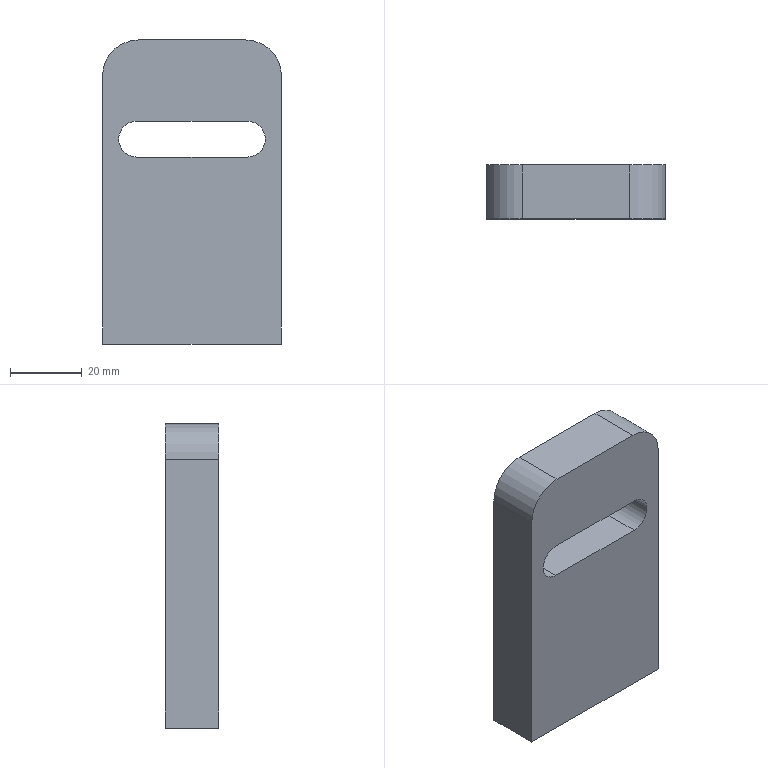Component | NX | BRACKET_2 | 1 solid | 22 faces | volume 56045 mm3 | plane 10 | cylinder 8 | cone 4 | commonest cylinder face diameters 10 x4 20 x2 6.8 x2